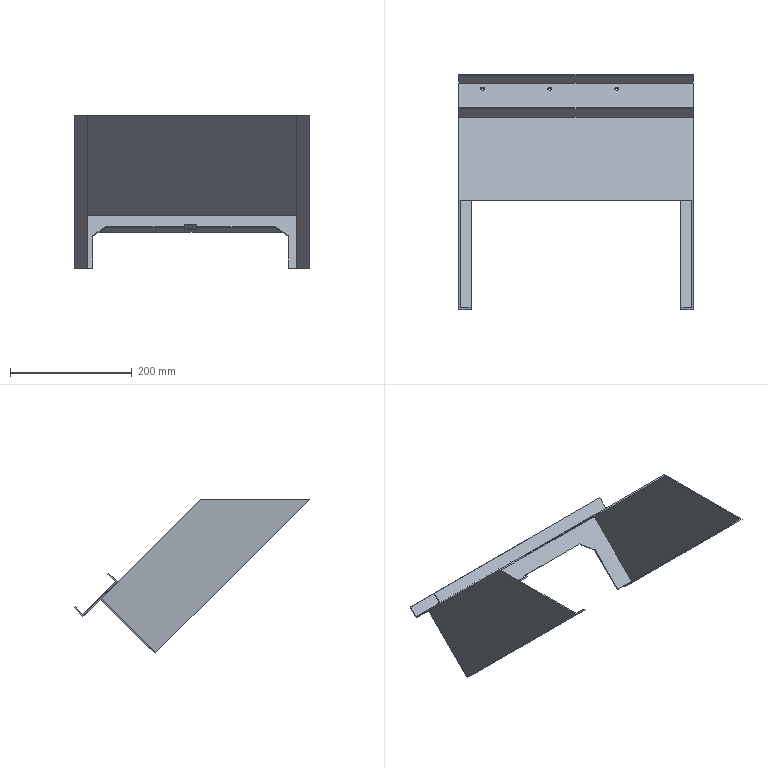Component | SolidWorks | GeneralAssembly-1_3-1 | 3 solids | 52 faces | box 384 x 386.08 x 252.44 mm | volume 474061 mm3 | plane 44 | cylinder 8 | commonest cylinder face diameters 7 x6 6 x2
build123d program:
from build123d import *

# Parameters (mm, degrees)
EXTRUDE_THIN1_DEPTH = 230
BOSS_EXTRUDE1_DEPTH = 2
BOSS_EXTRUDE2_DEPTH = 2
SKETCH4_W           = 18
SKETCH4_H           = 2
BOSS_EXTRUDE3_DEPTH = 127
CUT_EXTRUDE1_DEPTH  = 380
BOSS_EXTRUDE4_DEPTH = 2
EXTRUDE_THIN4_DEPTH = 384
SKETCH8_W           = 20
SKETCH8_H           = 10
BOSS_EXTRUDE5_DEPTH = 4
SKETCH9_W           = 8
SKETCH9_H           = 2
CUT_EXTRUDE2_DEPTH  = 20
SKETCH10_R          = 3
CUT_EXTRUDE3_DEPTH  = 2
SKETCH11_R          = 3.5
CUT_EXTRUDE4_DEPTH  = 10


with BuildPart() as part:
    # Sketch1 → Extrude-Thin1 (new body)
    with BuildSketch(Plane.XY):
        Polygon((-34.552, -105.631), (-54.552, -105.631), (-54.552, 21.369), (329.448, 21.369), (329.448, -105.631), (309.448, -105.631), (309.448, -103.631), (327.448, -103.631), (327.448, 19.369), (-52.552, 19.369), (-52.552, -103.631), (-34.552, -103.631), align=None)
    extrude(amount=EXTRUDE_THIN1_DEPTH)

    # Sketch2 → Boss-Extrude1 (add)
    with BuildSketch(Plane(origin=(329.448, 0, 0), x_dir=(0, 0, -1), z_dir=(1, 0, 0))):
        Polygon((-230, 21.369), (-357, -105.631), (-230, -105.631), align=None)
    extrude(amount=-BOSS_EXTRUDE1_DEPTH)

    # Sketch3 → Boss-Extrude2 (add)
    with BuildSketch(Plane.ZY.offset(54.552)):
        Polygon((230, 21.369), (357, -105.631), (230, -105.631), align=None)
    extrude(amount=-BOSS_EXTRUDE2_DEPTH)

    # Sketch4 → Boss-Extrude3 (add)
    with BuildSketch(Plane.XY.offset(230)):
        with Locations((-43.552, -104.631)):
            Rectangle(SKETCH4_W, SKETCH4_H)
        with Locations((318.448, -104.631)):
            Rectangle(SKETCH4_W, SKETCH4_H)
    extrude(amount=BOSS_EXTRUDE3_DEPTH)

    # Sketch5 → Cut-Extrude1 (cut)
    with BuildSketch(Plane.ZY.offset(52.552)):
        Polygon((355, -103.631), (357, -103.631), (357, -105.631), align=None)
    extrude(amount=-CUT_EXTRUDE1_DEPTH, mode=Mode.SUBTRACT)


with BuildPart() as body_2:
    # Sketch6 → Boss-Extrude4 (new body)
    with BuildSketch(Plane(origin=(0, 0, 0), x_dir=(-1, 0, 0), z_dir=(0, 0, -1))):
        Polygon((-295.448, -103.631), (-329.448, -103.631), (-329.448, 21.369), (54.552, 21.369), (54.552, -103.631), (25.552, -103.631), (25.552, -28.631), (4.552, -7.631), (-274.448, -7.631), (-295.448, -28.631), align=None)
    extrude(amount=BOSS_EXTRUDE4_DEPTH)

    # Sketch8 → Boss-Extrude5 (add)
    with BuildSketch(Plane.XZ.offset(7.631)):
        with Locations((134.948, 3)):
            Rectangle(SKETCH8_W, SKETCH8_H)
    extrude(amount=BOSS_EXTRUDE5_DEPTH)

    # Sketch9 → Cut-Extrude2 (cut)
    with BuildSketch(Plane.ZY.offset(-124.948)):
        with Locations((4, -8.631)):
            Rectangle(SKETCH9_W, SKETCH9_H)
    extrude(amount=-CUT_EXTRUDE2_DEPTH, mode=Mode.SUBTRACT)

    # Sketch10 → Cut-Extrude3 (cut)
    with BuildSketch(Plane(origin=(0, -11.631, 0), x_dir=(-1, 0, 0), z_dir=(0, -1, 0))):
        with Locations(Location((-134.948, -3, 0), (0, 0, 180))):
            Circle(SKETCH10_R)
    extrude(amount=-CUT_EXTRUDE3_DEPTH, mode=Mode.SUBTRACT)


with BuildPart() as body_3:
    # Sketch7 → Extrude-Thin4 (new body)
    with BuildSketch(Plane(origin=(329.448, 0, 0), x_dir=(0, 0, -1), z_dir=(1, 0, 0))):
        Polygon((-38, 41.369), (-38, 21.369), (42, 21.369), (42, 41.369), (40, 41.369), (40, 23.369), (-36, 23.369), (-36, 41.369), align=None)
    extrude(amount=-EXTRUDE_THIN4_DEPTH)

    # Sketch11 → Cut-Extrude4 (cut)
    with BuildSketch(Plane(origin=(0, 21.369, 0), x_dir=(-1, 0, 0), z_dir=(0, -1, 0))):
        with Locations(Location((15.552, 27, 0), (0, 0, 90))):
            Circle(SKETCH11_R)
        with Locations(Location((-94.448, 27, 0), (0, 0, 90))):
            Circle(SKETCH11_R)
        with Locations(Location((-204.448, 27, 0), (0, 0, 90))):
            Circle(SKETCH11_R)
    extrude(amount=-CUT_EXTRUDE4_DEPTH, mode=Mode.SUBTRACT)


solid = Compound([part.part, body_2.part, body_3.part])

# Placed as in the assembly
solid = solid.moved(Location((24.377, 418.31, -538.243), (45, 0, 0)))